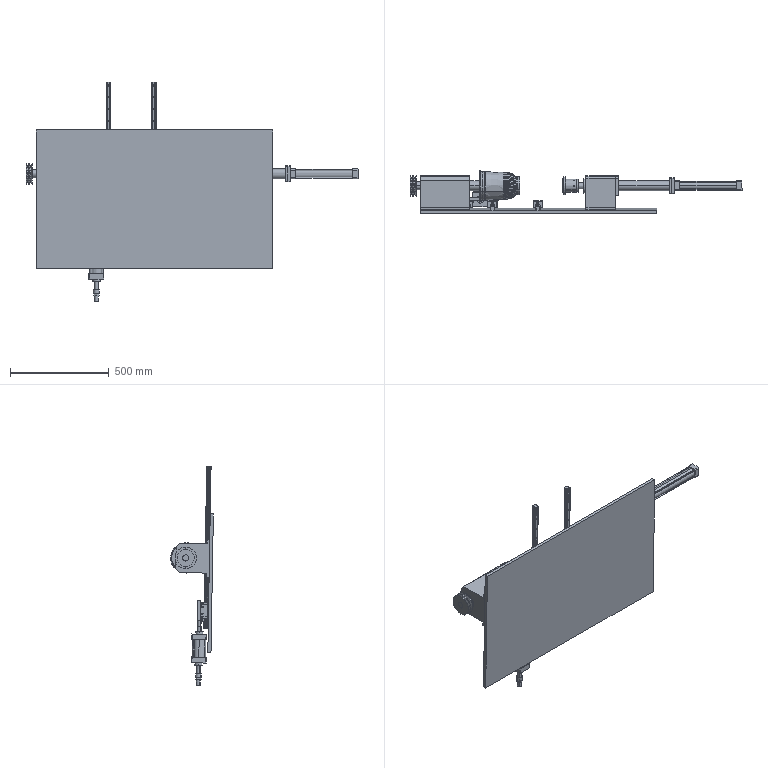Assembly | SolidWorks | mm | 29 component files | 29 solids | 1813 faces | box 1682.75 x 216.79 x 1111.76 mm | volume 26252304 mm3 | plane 606 | cylinder 569 | torus 412 | cone 150 | sphere 76 | commonest cylinder face diameters 11 x88 7 x80 6 x56 1 x24 5 x24 4.6 x20 6.6 x16 9 x16
Bill of materials:
30LinearBearing | 2 |  | Flanged cylindrical sleeve: a circular flange with four through holes at one end of a plain cylindrical hub with a through bore.
Axis | 1 |  | Long stepped round shaft with a thin disc collar near one end and a short small-diameter pin sticking out past the collar.
BearingHousing | 1 |  | Rectangular block with a plate-like flange lip at one end. A large round bore runs through one side face, and the end profile has two chamfered corners.
CutterFrontAndRearMovingPlate | 1 |  | Flat rectangular plate with eight through holes arranged in two 2x2 groups, one near each short end.
CylinderPlate | 1 |  | Square plate with small chamfered corners, a large central through hole, four larger holes near the corners, and four smaller holes on an inner square pattern.
CylinderSeat | 1 |  | Long hollow tube with a square flange plate at each end. Each flange has four corner holes, and the two flanges are different sizes.
deep groove ball bearings gb 16005 | 2 |  | Ring-shaped rolling-element assembly: an outer ring and an inner ring separated by a single row of spherical balls. It resembles an open ball bearing.
EdgeTrimmingTableSLDPRT | 1 | Plain Carbon Steel | Thin flat rectangular sheet or panel with no visible holes or features.
EdgeTrimmingWorkpiece | 1 |  | Hollow, bottle- or bullet-shaped thin-walled shell. A slightly tapered main body rounds into a smaller cylindrical neck, and the large open end has a thin flange lip.
EdgeTrimmingWorkpieceMold | 1 |  | Rounded, bullet-shaped body that narrows at the shoulder into a short cylindrical neck with an open bore. It is similar in form to the flanged shell but has no flange lip.
HGH25CAGuideRail(FrontAndRear) | 2 |  | Very long slender straight profile bar with a row of evenly spaced holes along its top face. Its cross-section has grooves along both sides.
HGH25CASlider | 3 |  | Rectangular block with an inverted, roughly U-shaped channel along its underside, grooved channel walls, chamfered corners, a thinner end-plate layer, and small holes on the end and side faces.
MoldMountingPlate | 1 |  | Thin circular disc with a small central through-hole and a shallow raised step of slightly smaller diameter on one face (stepped washer/disc shape).
PressHeadBearingHousing | 1 |  | Thick-walled cylindrical sleeve with a large through-bore. The visible end face has a counterbore or step at the bore and six small holes evenly spaced around it.
PressurePlate | 1 |  | Headed pin: a solid cylindrical shank with a short larger-diameter collar, a large thin circular head flange, and a slightly smaller thin disc layer behind the head.
SC40-200PistonRod | 1 | Plain Carbon Steel | Long slender solid cylindrical rod with a reduced-diameter stepped section at one end.
SC40-250Cylinder | 1 |  | Elongated assembly-like body: a central cylindrical barrel held between two square blocks with rounded corners at the ends. Thin rods run along the barrel, and a short cylindrical boss projects from one end block.
SC63-50Cylinder | 1 |  | Compact body: two square end blocks with chamfered corners around a central cylindrical barrel, with thin rods at the corners. Short cylindrical bosses project from both ends, and the top boss has a central hole.
SC63-50CylinderAxis | 1 |  | Slender stepped shaft or pin: a long main cylindrical section, a smaller-diameter tip at one end, and a short larger collar near the other end followed by a reduced-diameter stub.
Tailstock | 1 |  | Box-shaped block bracket: a rectangular body with a thin flange plate on one end that extends beyond the body. The flange has four corner holes, and a large round through-hole passes through the side faces. The far end has chamfered corners.
TailstockAxis | 1 |  | Long tube or shaft with a circular flange at one end. The flange has six evenly spaced holes. A long through-slot runs along part of the shaft, and the free end shows a small central bore.
tapered roller bearings gb 40x80x18.25 | 2 |  | Annular ring assembly shaped like a rolling-element bearing: an outer ring, an inner ring, and a single row of cylindrical rollers between them. The inner ring projects axially beyond the outer ring on one side.
TypeAPulley(Motor) | 1 |  | Circular sheave or pulley with two V-shaped circumferential grooves around its rim and a central through-bore.
Mates:
1. coincident | EdgeTrimmingTableSLDPRT-1 face at (877.004, 1175.798, 909.987) dir (0, 0.9998, 0.01745) | BearingHousing-1 face at (-322.996, 1181.033, 610.033) dir (0, -0.9998, -0.01745)
2. concentric | BearingHousing-1 face at (-90.996, 1299.706, 687.116) dir (1, 0, 0) r 40 | tapered roller bearings gb 40x80x18.25-2 face at (-72.743, 1299.706, 687.116) dir (-1, 0, 0) r 40
3. coincident | BearingHousing-1 face at (-90.996, 1299.706, 687.116) dir (1, 0, 0) | tapered roller bearings gb 40x80x18.25-2 face at (-90.996, 1338.706, 687.116) dir (-1, 0, 0)
4. concentric | BearingHousing-1 face at (-304.996, 1299.706, 687.116) dir (-1, 0, 0) r 40 | tapered roller bearings gb 40x80x18.25-1 face at (-323.249, 1299.706, 687.116) dir (1, 0, 0) r 40
5. coincident | BearingHousing-1 face at (-304.996, 1299.706, 687.116) dir (-1, 0, 0) | tapered roller bearings gb 40x80x18.25-1 face at (-304.996, 1334.677, 669.853) dir (1, 0, 0)
6. concentric | tapered roller bearings gb 40x80x18.25-2 face at (-72.743, 1299.706, 687.116) dir (-1, 0, 0) r 20 | Axis-1 face at (-537.368, 1299.706, 687.116) dir (-1, 0, 0) r 19.9
7. coincident | tapered roller bearings gb 40x80x18.25-2 face at (-72.743, 1299.706, 687.116) dir (1, 0, 0) | Axis-1 face at (-72.743, 1319.706, 687.116) dir (-1, 0, 0)
8. distance | BearingHousing-1 face at (-322.996, 1348.389, 762.977) dir (0, -0.01745, 0.9998) | EdgeTrimmingTableSLDPRT-1 face at (-322.996, 1175.798, 909.987) dir (0, -0.01745, 0.9998)
9. concentric | Axis-1 face at (-537.368, 1299.706, 687.116) dir (-1, 0, 0) r 50 | MoldMountingPlate-1 face at (-6.743, 1299.706, 687.116) dir (-1, 0, 0) r 71.765
10. coincident | Axis-1 face at (-6.743, 1349.706, 687.116) dir (1, 0, 0) | MoldMountingPlate-1 face at (-6.743, 1371.471, 687.116) dir (-1, 0, 0)
11. concentric | EdgeTrimmingWorkpieceMold-1 face at (6.082, 1299.706, 687.116) dir (1, 0, 0) r 34.907 | MoldMountingPlate-1 face at (-6.743, 1299.706, 687.116) dir (-1, 0, 0) r 71.765
12. coincident | EdgeTrimmingWorkpieceMold-1 face at (1.257, 1365.511, 715.758) dir (-1, 0, 0) | MoldMountingPlate-1 face at (1.257, 1361.471, 687.116) dir (1, 0, 0)
13. coincident | EdgeTrimmingWorkpieceMold-1 face at (98.626, 1299.706, 687.116) dir (1, 0, 0) r 34.907 | EdgeTrimmingWorkpiece-2 face at (6.257, 1299.706, 687.116) dir (1, 0, 0) r 34.907
14. concentric | PressurePlate-1 face at (411.936, 1299.706, 687.116) dir (-1, 0, 0) r 45 | PressHeadBearingHousing-1 face at (432.936, 1299.706, 687.116) dir (-1, 0, 0) r 32.5
15. concentric | Axis-1 face at (-537.368, 1299.706, 687.116) dir (-1, 0, 0) r 25 | PressHeadBearingHousing-1 face at (432.936, 1299.706, 687.116) dir (-1, 0, 0) r 32.5
16. coincident | EdgeTrimmingTableSLDPRT-1 face at (877.004, 1175.798, 909.987) dir (0, 0.9998, 0.01745) | Tailstock-1 face at (517.004, 1178.503, 755.011) dir (0, -0.9998, -0.01745)
17. concentric | PressHeadBearingHousing-1 face at (453.936, 1299.706, 687.116) dir (1, 0, 0) r 23.5 | deep groove ball bearings gb 16005-4 face at (466.647, 1299.706, 687.116) dir (1, 0, 0) r 23.5
18. coincident | PressHeadBearingHousing-1 face at (453.936, 1299.706, 687.116) dir (1, 0, 0) | deep groove ball bearings gb 16005-4 face at (453.936, 1308.967, 665.518) dir (-1, 0, 0)
19. concentric | deep groove ball bearings gb 16005-3 face at (414.226, 1299.706, 687.116) dir (-1, 0, 0) r 23.5 | PressHeadBearingHousing-1 face at (426.936, 1299.706, 687.116) dir (-1, 0, 0) r 23.5
20. coincident | deep groove ball bearings gb 16005-3 face at (426.936, 1323.206, 687.116) dir (1, 0, 0) | PressHeadBearingHousing-1 face at (426.936, 1299.706, 687.116) dir (-1, 0, 0)
21. coincident | deep groove ball bearings gb 16005-3 face at (418.936, 1315.873, 687.116) dir (-1, 0, 0) | PressurePlate-1 face at (418.936, 1299.706, 687.116) dir (1, 0, 0)
22. concentric | Tailstock-1 face at (517.004, 1299.706, 687.116) dir (1, 0, 0) r 22.5 | TailstockAxis-1 face at (432.161, 1299.706, 687.116) dir (-1, 0, 0) r 15
23. concentric | PressHeadBearingHousing-1 face at (432.936, 1299.706, 687.116) dir (-1, 0, 0) r 32.5 | TailstockAxis-1 face at (432.161, 1299.706, 687.116) dir (-1, 0, 0) r 32.5
24. coincident | PressHeadBearingHousing-1 face at (468.936, 1299.706, 687.116) dir (1, 0, 0) | TailstockAxis-1 face at (468.936, 1299.296, 710.612) dir (-1, 0, 0)
25. concentric | PressHeadBearingHousing-1 face at (453.936, 1275.217, 700.691) dir (1, 0, 0) r 2.1 | TailstockAxis-1 face at (488.936, 1275.217, 700.691) dir (-1, 0, 0) r 3
26. concentric | Tailstock-1 face at (517.004, 1299.706, 687.116) dir (1, 0, 0) r 22.5 | 30LinearBearing-1 face at (446.433, 1299.706, 687.116) dir (-1, 0, 0) r 22.5
27. coincident | Tailstock-1 face at (517.004, 1179.724, 685.022) dir (-1, 0, 0) | 30LinearBearing-1 face at (517.004, 1329.182, 709.481) dir (1, 0, 0)
28. concentric | Tailstock-1 face at (517.004, 1299.706, 687.116) dir (1, 0, 0) r 22.5 | 30LinearBearing-2 face at (737.575, 1299.706, 687.116) dir (1, 0, 0) r 22.5
29. coincident | Tailstock-1 face at (667.004, 1179.724, 685.022) dir (1, 0, 0) | 30LinearBearing-2 face at (667.004, 1322.071, 657.64) dir (-1, 0, 0)
30. concentric | 30LinearBearing-1 face at (513.504, 1323.605, 705.25) dir (-1, 0, 0) r 5.5 | 30LinearBearing-2 face at (670.504, 1323.605, 705.25) dir (1, 0, 0) r 5.5
31. concentric | SC40-200PistonRod-1 face at (921.936, 1299.706, 687.116) dir (1, 0, 0) r 8 | SC40-250Cylinder-1 face at (1050.004, 1299.706, 687.116) dir (-1, 0, 0) r 8
32. concentric | TailstockAxis-1 face at (432.161, 1299.706, 687.116) dir (-1, 0, 0) r 15 | CylinderSeat-1 face at (683.004, 1299.706, 687.116) dir (-1, 0, 0) r 20
33. coincident | Tailstock-1 face at (517.004, 1190.85, 735.223) dir (0, -0.01745, 0.9998) | CylinderSeat-1 face at (667.004, 1348.826, 737.981) dir (0, -0.01745, 0.9998)
34. coincident | Tailstock-1 face at (667.004, 1179.724, 685.022) dir (1, 0, 0) | CylinderSeat-1 face at (667.004, 1299.706, 687.116) dir (-1, 0, 0)
35. distance | SC40-200PistonRod-1 face at (897.936, 1299.706, 687.116) dir (-1, 0, 0) | SC40-250Cylinder-1 face at (950.004, 1299.706, 687.116) dir (-1, 0, 0)
36. concentric | SC40-250Cylinder-1 face at (950.004, 1299.706, 687.116) dir (1, 0, 0) r 16 | CylinderSeat-1 face at (683.004, 1299.706, 687.116) dir (-1, 0, 0) r 20
37. parallel | SC40-250Cylinder-1 face at (965.004, 1325.139, 662.556) dir (0, 0.9998, 0.01745) | CylinderSeat-1 face at (953.004, 1339.002, 727.808) dir (0, 0.9998, 0.01745)
38. distance | 30LinearBearing-1 face at (507.004, 1311.656, 696.183) dir (-1, 0, 0) | TailstockAxis-1 face at (478.936, 1299.139, 719.611) dir (1, 0, 0)
39. distance | Tailstock-1 face at (517.004, 1179.724, 685.022) dir (-1, 0, 0) | BearingHousing-1 face at (-72.996, 1264.711, 686.505) dir (1, 0, 0)
40. distance | SC40-200PistonRod-1 face at (921.936, 1299.706, 687.116) dir (-1, 0, 0) | TailstockAxis-1 face at (911.936, 1299.444, 702.114) dir (1, 0, 0)
41. concentric | SC40-250Cylinder-1 face at (950.004, 1299.706, 687.116) dir (1, 0, 0) r 16 | CylinderPlate-1 face at (965.004, 1299.706, 687.116) dir (-1, 0, 0) r 16
42. concentric | SC40-250Cylinder-1 face at (1316.489, 1317.88, 705.936) dir (-1, 0, 0) r 3 | CylinderPlate-1 face at (965.004, 1317.88, 705.936) dir (-1, 0, 0) r 3.5
43. coincident | SC40-250Cylinder-1 face at (965.004, 1299.706, 687.116) dir (-1, 0, 0) | CylinderPlate-1 face at (965.004, 1299.706, 687.116) dir (1, 0, 0)
44. coincident | CylinderSeat-1 face at (953.004, 1299.706, 687.116) dir (1, 0, 0) | CylinderPlate-1 face at (953.004, 1299.706, 687.116) dir (-1, 0, 0)
45. coincident | HGH25CAGuideRail(FrontAndRear)-1 face at (264.954, 1183.54, 1151.159) dir (-1, 0, 0) | HGH25CASlider-5 face at (264.954, 1195.669, 456.249) dir (1, 0, 0)
46. coincident | HGH25CAGuideRail(FrontAndRear)-1 face at (273.004, 1193.588, 1151.335) dir (0, 0.9998, 0.01745) | HGH25CASlider-5 face at (261.504, 1207.245, 368.954) dir (0, -0.9998, -0.01745)
47. coincident | EdgeTrimmingTableSLDPRT-1 face at (877.004, 1175.798, 909.987) dir (0, 0.9998, 0.01745) | HGH25CAGuideRail(FrontAndRear)-1 face at (273.004, 1171.591, 1150.951) dir (0, -0.9998, -0.01745)
48. concentric | SC63-50Cylinder-1 face at (-17.996, 1231.175, 315.863) dir (0, 0.01745, -0.9998) r 19 | SC63-50CylinderAxis-1 face at (-17.996, 1230.2, 371.699) dir (0, -0.01745, 0.9998) r 10
49. distance | SC63-50CylinderAxis-1 face at (-17.996, 1230.2, 371.699) dir (0, -0.01745, 0.9998) | SC63-50Cylinder-1 face at (-17.996, 1231.175, 315.863) dir (0, -0.01745, 0.9998)
50. coincident | assembly face at (72.004, 1225.434, 358.264) dir (0, 0.01745, -0.9998) | SC63-50CylinderAxis-1 face at (-17.996, 1230.2, 371.699) dir (0, -0.01745, 0.9998)
51. coincident | HGH25CAGuideRail(FrontAndRear)-3 face at (43.004, 1193.588, 1151.335) dir (0, 0.9998, 0.01745) | HGH25CASlider-9 face at (31.504, 1207.003, 382.795) dir (0, -0.9998, -0.01745)
52. coincident | HGH25CAGuideRail(FrontAndRear)-3 face at (54.504, 1207.899, 331.46) dir (1, 0, 0) | HGH25CASlider-9 face at (54.504, 1185.006, 382.411) dir (-1, 0, 0)
53. concentric | HGH25CASlider-9 face at (60.504, 1224.634, 404.106) dir (0, 0.9998, 0.01745) r 3 | CutterFrontAndRearMovingPlate-3 face at (60.504, 1240.631, 404.386) dir (0, -0.9998, -0.01745) r 3.5
54. concentric | HGH25CASlider-9 face at (60.504, 1224.023, 439.101) dir (0, 0.9998, 0.01745) r 3 | CutterFrontAndRearMovingPlate-3 face at (60.504, 1240.021, 439.38) dir (0, -0.9998, -0.01745) r 3.5
55. coincident | HGH25CASlider-9 face at (19.004, 1222.791, 509.703) dir (0, 0.9998, 0.01745) | CutterFrontAndRearMovingPlate-3 face at (-17.996, 1224.328, 421.604) dir (0, -0.9998, -0.01745)
56. coincident | SC63-50CylinderAxis-1 face at (-17.996, 1230.2, 371.699) dir (0, -0.01745, 0.9998) | CutterFrontAndRearMovingPlate-3 face at (72.004, 1225.201, 371.611) dir (0, 0.01745, -0.9998)
57. concentric | Axis-1 face at (-537.368, 1299.706, 687.116) dir (-1, 0, 0) r 16 | TypeAPulley(Motor)-2 face at (-433.348, 1299.706, 687.116) dir (-1, 0, 0) r 16
58. coincident | Axis-1 face at (-342.743, 1315.706, 687.116) dir (-1, 0, 0) | TypeAPulley(Motor)-2 face at (-342.743, 1354.706, 687.116) dir (1, 0, 0)
59. coincident | EdgeTrimmingTableSLDPRT-1 face at (-322.996, 1188.014, 210.094) dir (-1, 0, 0) | BearingHousing-1 face at (-322.996, 1264.711, 686.505) dir (-1, 0, 0)
60. parallel | Tailstock-1 face at (517.004, 1190.85, 735.223) dir (0, -0.01745, 0.9998) | TailstockAxis-1 face at (568.936, 1319.773, 683.466) dir (0, -0.01745, 0.9998)